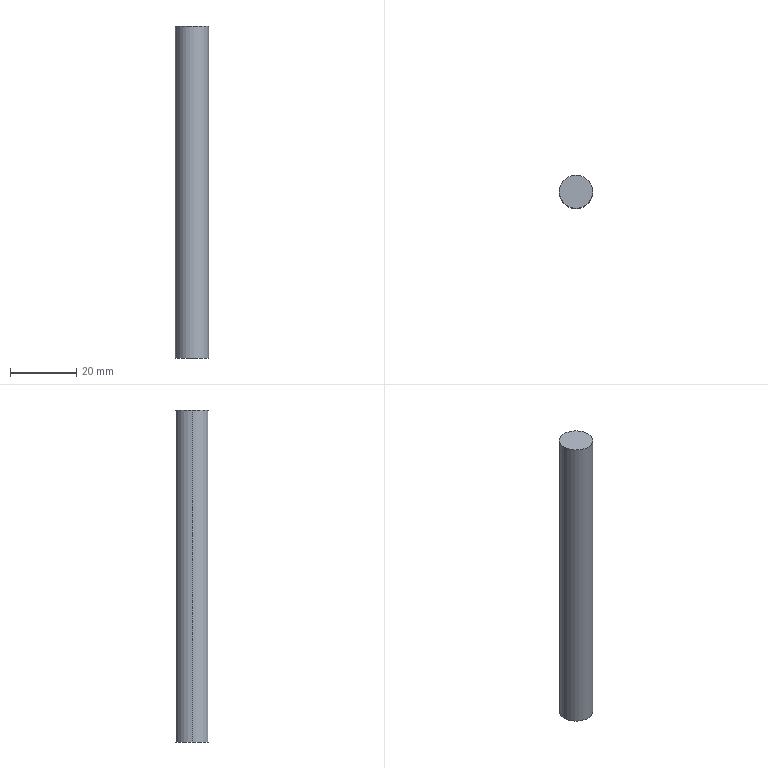Component | SolidWorks | CenterAxis-1 | 1 solid | 4 faces | box 10 x 10 x 100 mm | volume 7854 mm3 | cylinder 2 | plane 2 | commonest cylinder face diameters 10 x2
build123d program:
from build123d import *

# Parameters (mm, degrees)
SKETCH1_R           = 5
BOSS_EXTRUDE1_DEPTH = 100


with BuildPart() as part:
    # Sketch1 → Boss-Extrude1 (new body)
    with BuildSketch(Plane.XY):
        Circle(SKETCH1_R)
    extrude(amount=BOSS_EXTRUDE1_DEPTH)


solid = part.part

# Placed as in the assembly
solid = solid.moved(Location((1.903, -27.983, -2.5), (0, 0, 0)))
STEP:
#1=COLOUR_RGB('',0.7922,0.8196,0.9333);
#2=FILL_AREA_STYLE_COLOUR('',#1);
#3=FILL_AREA_STYLE('',(#2));
#4=SURFACE_STYLE_FILL_AREA(#3);
#5=SURFACE_SIDE_STYLE('',(#4));
#6=SURFACE_STYLE_USAGE(.BOTH.,#5);
#7=PRESENTATION_STYLE_ASSIGNMENT((#6));
#8=CARTESIAN_POINT('',(0.2718,-1.102,3.839));
#9=VERTEX_POINT('',#8);
#10=CARTESIAN_POINT('',(-0.1219,-1.102,3.839));
#11=VERTEX_POINT('',#10);
#12=CARTESIAN_POINT('',(0.07493,-1.102,3.839));
#13=DIRECTION('',(0.,0.,1.));
#14=DIRECTION('',(1.,0.,0.));
#15=AXIS2_PLACEMENT_3D('',#12,#13,#14);
#16=CIRCLE('',#15,0.1969);
#17=EDGE_CURVE('',#9,#11,#16,.T.);
#18=ORIENTED_EDGE('',*,*,#17,.F.);
#19=CARTESIAN_POINT('',(0.2718,-1.102,-0.09843));
#20=VERTEX_POINT('',#19);
#21=CARTESIAN_POINT('',(0.2718,-1.102,3.839));
#22=DIRECTION('',(0.,0.,-1.));
#23=VECTOR('',#22,39.37);
#24=LINE('',#21,#23);
#25=EDGE_CURVE('',#9,#20,#24,.T.);
#26=ORIENTED_EDGE('',*,*,#25,.T.);
#27=CARTESIAN_POINT('',(-0.1219,-1.102,-0.09843));
#28=VERTEX_POINT('',#27);
#29=CARTESIAN_POINT('',(0.07493,-1.102,-0.09843));
#30=DIRECTION('',(0.,0.,1.));
#31=DIRECTION('',(1.,0.,0.));
#32=AXIS2_PLACEMENT_3D('',#29,#30,#31);
#33=CIRCLE('',#32,0.1969);
#34=EDGE_CURVE('',#20,#28,#33,.T.);
#35=ORIENTED_EDGE('',*,*,#34,.T.);
#36=CARTESIAN_POINT('',(-0.1219,-1.102,3.839));
#37=DIRECTION('',(0.,0.,-1.));
#38=VECTOR('',#37,39.37);
#39=LINE('',#36,#38);
#40=EDGE_CURVE('',#11,#28,#39,.T.);
#41=ORIENTED_EDGE('',*,*,#40,.F.);
#42=EDGE_LOOP('',(#18,#26,#35,#41));
#43=FACE_OUTER_BOUND('',#42,.T.);
#44=CARTESIAN_POINT('',(0.07493,-1.102,3.839));
#45=DIRECTION('',(0.,0.,-1.));
#46=DIRECTION('',(-1.,0.,0.));
#47=AXIS2_PLACEMENT_3D('',#44,#45,#46);
#48=CYLINDRICAL_SURFACE('',#47,0.1969);
#49=ADVANCED_FACE('',(#43),#48,.T.);
#50=ORIENTED_EDGE('',*,*,#25,.F.);
#51=CARTESIAN_POINT('',(0.07493,-1.102,3.839));
#52=DIRECTION('',(0.,0.,1.));
#53=DIRECTION('',(1.,0.,0.));
#54=AXIS2_PLACEMENT_3D('',#51,#52,#53);
#55=CIRCLE('',#54,0.1969);
#56=EDGE_CURVE('',#11,#9,#55,.T.);
#57=ORIENTED_EDGE('',*,*,#56,.F.);
#58=ORIENTED_EDGE('',*,*,#40,.T.);
#59=CARTESIAN_POINT('',(0.07493,-1.102,-0.09843));
#60=DIRECTION('',(0.,0.,1.));
#61=DIRECTION('',(1.,0.,0.));
#62=AXIS2_PLACEMENT_3D('',#59,#60,#61);
#63=CIRCLE('',#62,0.1969);
#64=EDGE_CURVE('',#28,#20,#63,.T.);
#65=ORIENTED_EDGE('',*,*,#64,.T.);
#66=EDGE_LOOP('',(#50,#57,#58,#65));
#67=FACE_OUTER_BOUND('',#66,.T.);
#68=CARTESIAN_POINT('',(0.07493,-1.102,3.839));
#69=DIRECTION('',(0.,0.,-1.));
#70=DIRECTION('',(-1.,0.,0.));
#71=AXIS2_PLACEMENT_3D('',#68,#69,#70);
#72=CYLINDRICAL_SURFACE('',#71,0.1969);
#73=ADVANCED_FACE('',(#67),#72,.T.);
#74=ORIENTED_EDGE('',*,*,#56,.T.);
#75=ORIENTED_EDGE('',*,*,#17,.T.);
#76=EDGE_LOOP('',(#74,#75));
#77=FACE_OUTER_BOUND('',#76,.T.);
#78=CARTESIAN_POINT('',(0.07493,-1.102,3.839));
#79=DIRECTION('',(0.,0.,1.));
#80=DIRECTION('',(1.,0.,0.));
#81=AXIS2_PLACEMENT_3D('',#78,#79,#80);
#82=PLANE('',#81);
#83=ADVANCED_FACE('',(#77),#82,.T.);
#84=ORIENTED_EDGE('',*,*,#64,.F.);
#85=ORIENTED_EDGE('',*,*,#34,.F.);
#86=EDGE_LOOP('',(#84,#85));
#87=FACE_OUTER_BOUND('',#86,.T.);
#88=CARTESIAN_POINT('',(0.07493,-1.102,-0.09843));
#89=DIRECTION('',(0.,0.,1.));
#90=DIRECTION('',(1.,0.,0.));
#91=AXIS2_PLACEMENT_3D('',#88,#89,#90);
#92=PLANE('',#91);
#93=ADVANCED_FACE('',(#87),#92,.F.);
#94=CLOSED_SHELL('',(#49,#73,#83,#93));
#95=MANIFOLD_SOLID_BREP('',#94);
#96=STYLED_ITEM('',(#7),#95);
#97=PRESENTATION_LAYER_ASSIGNMENT('','',(#96));
#98=(LENGTH_UNIT()NAMED_UNIT(*)SI_UNIT($,.METRE.));
#99=LENGTH_MEASURE_WITH_UNIT(LENGTH_MEASURE(0.0254),#98);
#100=DIMENSIONAL_EXPONENTS(1.,0.,0.,0.,0.,0.,0.);
#101=(CONVERSION_BASED_UNIT('',#99)LENGTH_UNIT()NAMED_UNIT(#100));
#102=UNCERTAINTY_MEASURE_WITH_UNIT(LENGTH_MEASURE(0.00001),#101,'','');
#103=(NAMED_UNIT(*)PLANE_ANGLE_UNIT()SI_UNIT($,.RADIAN.));
#104=(NAMED_UNIT(*)SI_UNIT($,.STERADIAN.)SOLID_ANGLE_UNIT());
#105=(GEOMETRIC_REPRESENTATION_CONTEXT(3)GLOBAL_UNCERTAINTY_ASSIGNED_CONTEXT((#102))GLOBAL_UNIT_ASSIGNED_CONTEXT((#101,#103,#104))REPRESENTATION_CONTEXT('',''));
#106=MECHANICAL_DESIGN_GEOMETRIC_PRESENTATION_REPRESENTATION('',(#96),#105);
#107=CARTESIAN_POINT('',(0.,0.,0.));
#108=DIRECTION('',(0.,0.,1.));
#109=DIRECTION('',(1.,0.,0.));
#110=AXIS2_PLACEMENT_3D('',#107,#108,#109);
#111=(LENGTH_UNIT()NAMED_UNIT(*)SI_UNIT($,.METRE.));
#112=LENGTH_MEASURE_WITH_UNIT(LENGTH_MEASURE(0.0254),#111);
#113=DIMENSIONAL_EXPONENTS(1.,0.,0.,0.,0.,0.,0.);
#114=(CONVERSION_BASED_UNIT('',#112)LENGTH_UNIT()NAMED_UNIT(#113));
#115=UNCERTAINTY_MEASURE_WITH_UNIT(LENGTH_MEASURE(0.00001),#114,'','');
#116=(NAMED_UNIT(*)PLANE_ANGLE_UNIT()SI_UNIT($,.RADIAN.));
#117=(NAMED_UNIT(*)SI_UNIT($,.STERADIAN.)SOLID_ANGLE_UNIT());
#118=(GEOMETRIC_REPRESENTATION_CONTEXT(3)GLOBAL_UNCERTAINTY_ASSIGNED_CONTEXT((#115))GLOBAL_UNIT_ASSIGNED_CONTEXT((#114,#116,#117))REPRESENTATION_CONTEXT('',''));
#119=ADVANCED_BREP_SHAPE_REPRESENTATION('',(#95,#110),#118);